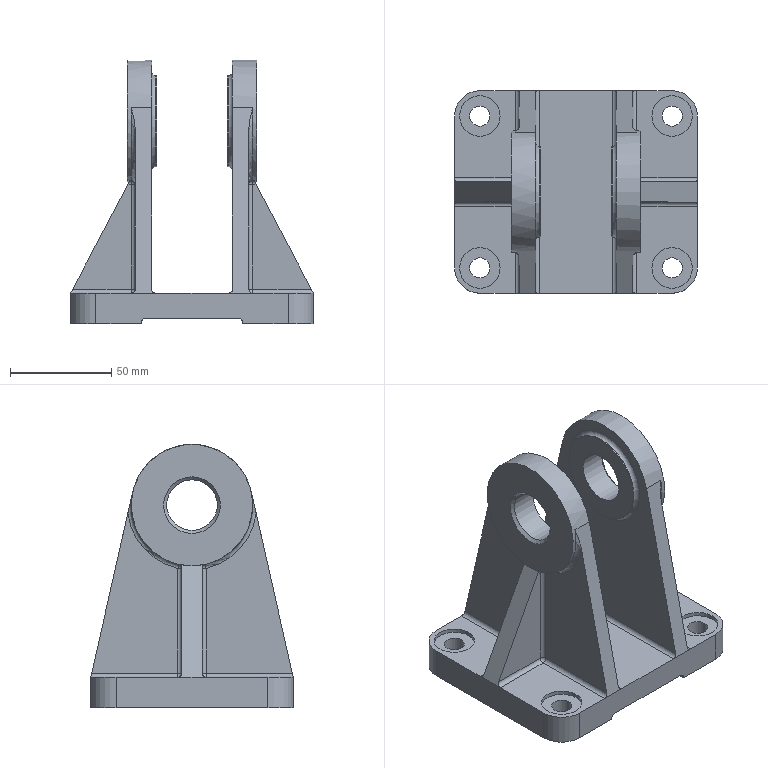Component | NX | 1_BRACKET | 1 solid | 92 faces | volume 328001 mm3 | plane 38 | cylinder 38 | sphere 8 | torus 6 | cone 2 | commonest cylinder face diameters 4 x20 25 x6 10 x4 20 x4 60 x2 45 x2